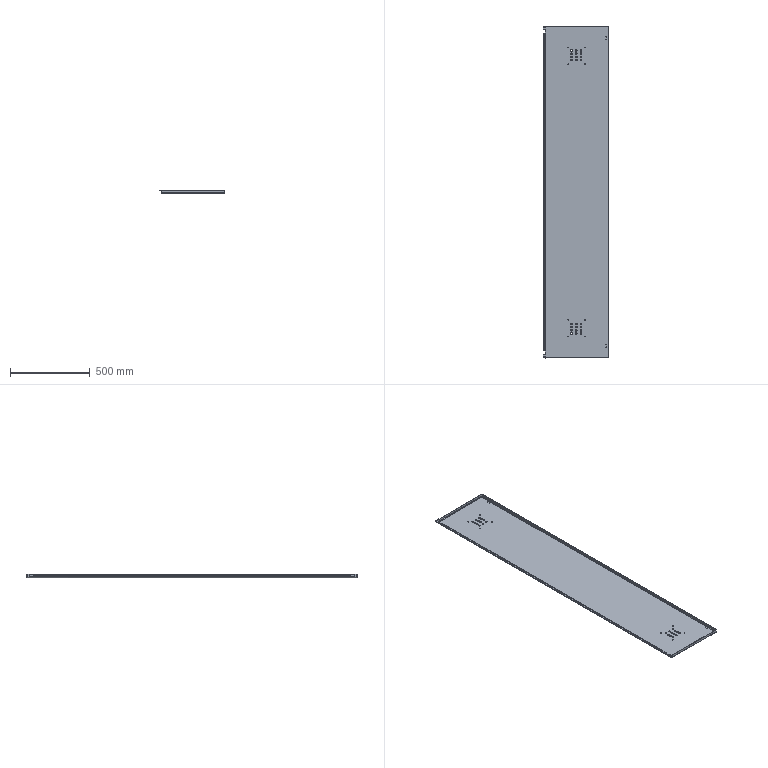Component | SolidWorks | LeftRearDoor-1_RearDoor1-1 | 1 solid | 146 faces | volume 1866049 mm3 | cylinder 86 | plane 52 | spline 8 | commonest cylinder face diameters 10 x48 5 x16 3.2 x8 11 x7 7 x7 | material Malleable Cast Iron